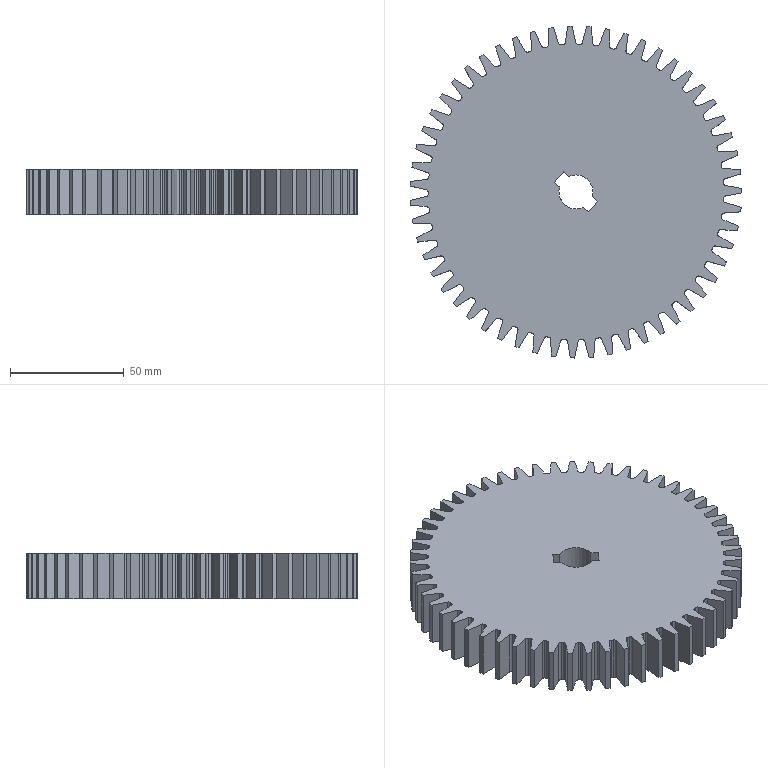Component | SolidWorks | SmallPulley1-4 | 1 solid | 366 faces | volume 291300 mm3 | cylinder 192 | plane 174 | commonest cylinder face diameters 2 x133 130 x55 3 x2 15 x2